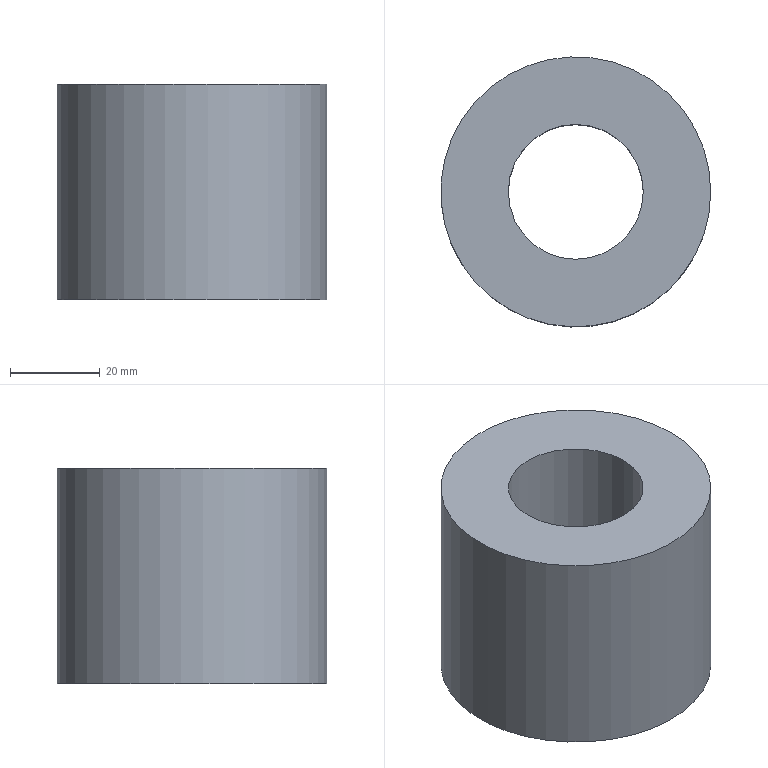Component | NX | CH3404_10-3 | 1 solid | 4 faces | box 60 x 60 x 48 mm | volume 101788 mm3 | cylinder 2 | plane 2 | commonest cylinder face diameters 60 x1 30 x1
STEP:
#1=CARTESIAN_POINT('',(0.,0.,0.));
#2=DIRECTION('',(0.,0.,1.));
#3=DIRECTION('',(1.,0.,0.));
#4=AXIS2_PLACEMENT_3D('',#1,#2,#3);
#5=CARTESIAN_POINT('',(30.,0.,130.));
#6=VERTEX_POINT('',#5);
#7=CARTESIAN_POINT('',(-0.,0.,130.));
#8=DIRECTION('',(0.,0.,1.));
#9=DIRECTION('',(1.,0.,0.));
#10=AXIS2_PLACEMENT_3D('',#7,#8,#9);
#11=CIRCLE('',#10,30.);
#12=CARTESIAN_POINT('',(-0.,0.,130.));
#13=DIRECTION('',(0.,0.,-1.));
#14=DIRECTION('',(-1.,0.,0.));
#15=AXIS2_PLACEMENT_3D('',#12,#13,#14);
#16=CYLINDRICAL_SURFACE('',#15,30.);
#17=CARTESIAN_POINT('',(9.425,0.));
#18=DIRECTION('',(-1.,0.));
#19=VECTOR('',#18,1.);
#20=LINE('',#17,#19);
#21=(GEOMETRIC_REPRESENTATION_CONTEXT(2)PARAMETRIC_REPRESENTATION_CONTEXT()REPRESENTATION_CONTEXT('',''));
#22=DEFINITIONAL_REPRESENTATION('',(#20),#21);
#23=PCURVE('',#16,#22);
#24=CARTESIAN_POINT('',(-0.,0.,130.));
#25=DIRECTION('',(0.,0.,1.));
#26=DIRECTION('',(1.,0.,0.));
#27=AXIS2_PLACEMENT_3D('',#24,#25,#26);
#28=PLANE('',#27);
#29=CARTESIAN_POINT('',(0.,0.));
#30=DIRECTION('',(1.,0.));
#31=AXIS2_PLACEMENT_2D('',#29,#30);
#32=CIRCLE('',#31,30.);
#33=(GEOMETRIC_REPRESENTATION_CONTEXT(2)PARAMETRIC_REPRESENTATION_CONTEXT()REPRESENTATION_CONTEXT('',''));
#34=DEFINITIONAL_REPRESENTATION('',(#32),#33);
#35=PCURVE('',#28,#34);
#36=SURFACE_CURVE('',#11,(#23,#35),.PCURVE_S1.);
#37=EDGE_CURVE('',#6,#6,#36,.T.);
#38=ORIENTED_EDGE('',*,*,#37,.F.);
#39=CARTESIAN_POINT('',(30.,0.,82.));
#40=VERTEX_POINT('',#39);
#41=CARTESIAN_POINT('',(30.,0.,130.));
#42=CARTESIAN_POINT('',(30.,0.,82.));
#43=B_SPLINE_CURVE_WITH_KNOTS('',1,(#41,#42),.UNSPECIFIED.,.F.,.F.,(2,2),(0.,48.),.PIECEWISE_BEZIER_KNOTS.);
#44=CARTESIAN_POINT('',(9.425,0.));
#45=DIRECTION('',(0.,1.));
#46=VECTOR('',#45,1.);
#47=LINE('',#44,#46);
#48=(GEOMETRIC_REPRESENTATION_CONTEXT(2)PARAMETRIC_REPRESENTATION_CONTEXT()REPRESENTATION_CONTEXT('',''));
#49=DEFINITIONAL_REPRESENTATION('',(#47),#48);
#50=PCURVE('',#16,#49);
#51=CARTESIAN_POINT('',(3.142,0.));
#52=DIRECTION('',(0.,1.));
#53=VECTOR('',#52,1.);
#54=LINE('',#51,#53);
#55=(GEOMETRIC_REPRESENTATION_CONTEXT(2)PARAMETRIC_REPRESENTATION_CONTEXT()REPRESENTATION_CONTEXT('',''));
#56=DEFINITIONAL_REPRESENTATION('',(#54),#55);
#57=PCURVE('',#16,#56);
#58=SEAM_CURVE('',#43,(#50,#57),.PCURVE_S1.);
#59=EDGE_CURVE('',#6,#40,#58,.T.);
#60=ORIENTED_EDGE('',*,*,#59,.T.);
#61=CARTESIAN_POINT('',(-0.,0.,82.));
#62=DIRECTION('',(0.,0.,1.));
#63=DIRECTION('',(1.,0.,0.));
#64=AXIS2_PLACEMENT_3D('',#61,#62,#63);
#65=CIRCLE('',#64,30.);
#66=CARTESIAN_POINT('',(9.425,48.));
#67=DIRECTION('',(-1.,0.));
#68=VECTOR('',#67,1.);
#69=LINE('',#66,#68);
#70=(GEOMETRIC_REPRESENTATION_CONTEXT(2)PARAMETRIC_REPRESENTATION_CONTEXT()REPRESENTATION_CONTEXT('',''));
#71=DEFINITIONAL_REPRESENTATION('',(#69),#70);
#72=PCURVE('',#16,#71);
#73=CARTESIAN_POINT('',(-0.,0.,82.));
#74=DIRECTION('',(0.,0.,1.));
#75=DIRECTION('',(1.,0.,0.));
#76=AXIS2_PLACEMENT_3D('',#73,#74,#75);
#77=PLANE('',#76);
#78=CARTESIAN_POINT('',(0.,0.));
#79=DIRECTION('',(1.,0.));
#80=AXIS2_PLACEMENT_2D('',#78,#79);
#81=CIRCLE('',#80,30.);
#82=(GEOMETRIC_REPRESENTATION_CONTEXT(2)PARAMETRIC_REPRESENTATION_CONTEXT()REPRESENTATION_CONTEXT('',''));
#83=DEFINITIONAL_REPRESENTATION('',(#81),#82);
#84=PCURVE('',#77,#83);
#85=SURFACE_CURVE('',#65,(#72,#84),.PCURVE_S1.);
#86=EDGE_CURVE('',#40,#40,#85,.T.);
#87=ORIENTED_EDGE('',*,*,#86,.T.);
#88=ORIENTED_EDGE('',*,*,#59,.F.);
#89=EDGE_LOOP('',(#38,#60,#87,#88));
#90=FACE_BOUND('',#89,.T.);
#91=ADVANCED_FACE('',(#90),#16,.T.);
#92=CARTESIAN_POINT('',(15.,0.,130.));
#93=VERTEX_POINT('',#92);
#94=CARTESIAN_POINT('',(-0.,0.,130.));
#95=DIRECTION('',(0.,0.,1.));
#96=DIRECTION('',(1.,0.,0.));
#97=AXIS2_PLACEMENT_3D('',#94,#95,#96);
#98=CIRCLE('',#97,15.);
#99=CARTESIAN_POINT('',(-0.,0.,130.));
#100=DIRECTION('',(0.,0.,-1.));
#101=DIRECTION('',(-1.,0.,0.));
#102=AXIS2_PLACEMENT_3D('',#99,#100,#101);
#103=CYLINDRICAL_SURFACE('',#102,15.);
#104=CARTESIAN_POINT('',(9.425,0.));
#105=DIRECTION('',(-1.,0.));
#106=VECTOR('',#105,1.);
#107=LINE('',#104,#106);
#108=(GEOMETRIC_REPRESENTATION_CONTEXT(2)PARAMETRIC_REPRESENTATION_CONTEXT()REPRESENTATION_CONTEXT('',''));
#109=DEFINITIONAL_REPRESENTATION('',(#107),#108);
#110=PCURVE('',#103,#109);
#111=CARTESIAN_POINT('',(0.,0.));
#112=DIRECTION('',(1.,0.));
#113=AXIS2_PLACEMENT_2D('',#111,#112);
#114=CIRCLE('',#113,15.);
#115=(GEOMETRIC_REPRESENTATION_CONTEXT(2)PARAMETRIC_REPRESENTATION_CONTEXT()REPRESENTATION_CONTEXT('',''));
#116=DEFINITIONAL_REPRESENTATION('',(#114),#115);
#117=PCURVE('',#28,#116);
#118=SURFACE_CURVE('',#98,(#110,#117),.PCURVE_S1.);
#119=EDGE_CURVE('',#93,#93,#118,.T.);
#120=ORIENTED_EDGE('',*,*,#119,.F.);
#121=CARTESIAN_POINT('',(15.,0.,82.));
#122=VERTEX_POINT('',#121);
#123=CARTESIAN_POINT('',(15.,0.,130.));
#124=CARTESIAN_POINT('',(15.,0.,82.));
#125=B_SPLINE_CURVE_WITH_KNOTS('',1,(#123,#124),.UNSPECIFIED.,.F.,.F.,(2,2),(0.,48.),.PIECEWISE_BEZIER_KNOTS.);
#126=CARTESIAN_POINT('',(9.425,0.));
#127=DIRECTION('',(0.,1.));
#128=VECTOR('',#127,1.);
#129=LINE('',#126,#128);
#130=(GEOMETRIC_REPRESENTATION_CONTEXT(2)PARAMETRIC_REPRESENTATION_CONTEXT()REPRESENTATION_CONTEXT('',''));
#131=DEFINITIONAL_REPRESENTATION('',(#129),#130);
#132=PCURVE('',#103,#131);
#133=CARTESIAN_POINT('',(3.142,0.));
#134=DIRECTION('',(0.,1.));
#135=VECTOR('',#134,1.);
#136=LINE('',#133,#135);
#137=(GEOMETRIC_REPRESENTATION_CONTEXT(2)PARAMETRIC_REPRESENTATION_CONTEXT()REPRESENTATION_CONTEXT('',''));
#138=DEFINITIONAL_REPRESENTATION('',(#136),#137);
#139=PCURVE('',#103,#138);
#140=SEAM_CURVE('',#125,(#132,#139),.PCURVE_S1.);
#141=EDGE_CURVE('',#93,#122,#140,.T.);
#142=ORIENTED_EDGE('',*,*,#141,.T.);
#143=CARTESIAN_POINT('',(-0.,0.,82.));
#144=DIRECTION('',(0.,0.,1.));
#145=DIRECTION('',(1.,0.,0.));
#146=AXIS2_PLACEMENT_3D('',#143,#144,#145);
#147=CIRCLE('',#146,15.);
#148=CARTESIAN_POINT('',(9.425,48.));
#149=DIRECTION('',(-1.,0.));
#150=VECTOR('',#149,1.);
#151=LINE('',#148,#150);
#152=(GEOMETRIC_REPRESENTATION_CONTEXT(2)PARAMETRIC_REPRESENTATION_CONTEXT()REPRESENTATION_CONTEXT('',''));
#153=DEFINITIONAL_REPRESENTATION('',(#151),#152);
#154=PCURVE('',#103,#153);
#155=CARTESIAN_POINT('',(0.,0.));
#156=DIRECTION('',(1.,0.));
#157=AXIS2_PLACEMENT_2D('',#155,#156);
#158=CIRCLE('',#157,15.);
#159=(GEOMETRIC_REPRESENTATION_CONTEXT(2)PARAMETRIC_REPRESENTATION_CONTEXT()REPRESENTATION_CONTEXT('',''));
#160=DEFINITIONAL_REPRESENTATION('',(#158),#159);
#161=PCURVE('',#77,#160);
#162=SURFACE_CURVE('',#147,(#154,#161),.PCURVE_S1.);
#163=EDGE_CURVE('',#122,#122,#162,.T.);
#164=ORIENTED_EDGE('',*,*,#163,.T.);
#165=ORIENTED_EDGE('',*,*,#141,.F.);
#166=EDGE_LOOP('',(#120,#142,#164,#165));
#167=FACE_BOUND('',#166,.F.);
#168=ADVANCED_FACE('',(#167),#103,.F.);
#169=ORIENTED_EDGE('',*,*,#37,.T.);
#170=EDGE_LOOP('',(#169));
#171=FACE_BOUND('',#170,.T.);
#172=ORIENTED_EDGE('',*,*,#119,.F.);
#173=EDGE_LOOP('',(#172));
#174=FACE_BOUND('',#173,.T.);
#175=ADVANCED_FACE('',(#171,#174),#28,.T.);
#176=ORIENTED_EDGE('',*,*,#86,.F.);
#177=EDGE_LOOP('',(#176));
#178=FACE_BOUND('',#177,.T.);
#179=ORIENTED_EDGE('',*,*,#163,.T.);
#180=EDGE_LOOP('',(#179));
#181=FACE_BOUND('',#180,.T.);
#182=ADVANCED_FACE('',(#178,#181),#77,.F.);
#183=CLOSED_SHELL('',(#91,#168,#175,#182));
#184=MANIFOLD_SOLID_BREP('',#183);
#185=(LENGTH_UNIT()NAMED_UNIT(*)SI_UNIT(.MILLI.,.METRE.));
#186=UNCERTAINTY_MEASURE_WITH_UNIT(LENGTH_MEASURE(0.00001),#185,'','');
#187=(NAMED_UNIT(*)PLANE_ANGLE_UNIT()SI_UNIT($,.RADIAN.));
#188=(NAMED_UNIT(*)SI_UNIT($,.STERADIAN.)SOLID_ANGLE_UNIT());
#189=(GEOMETRIC_REPRESENTATION_CONTEXT(3)GLOBAL_UNCERTAINTY_ASSIGNED_CONTEXT((#186))GLOBAL_UNIT_ASSIGNED_CONTEXT((#185,#187,#188))REPRESENTATION_CONTEXT('',''));
#190=ADVANCED_BREP_SHAPE_REPRESENTATION('',(#4,#184),#189);